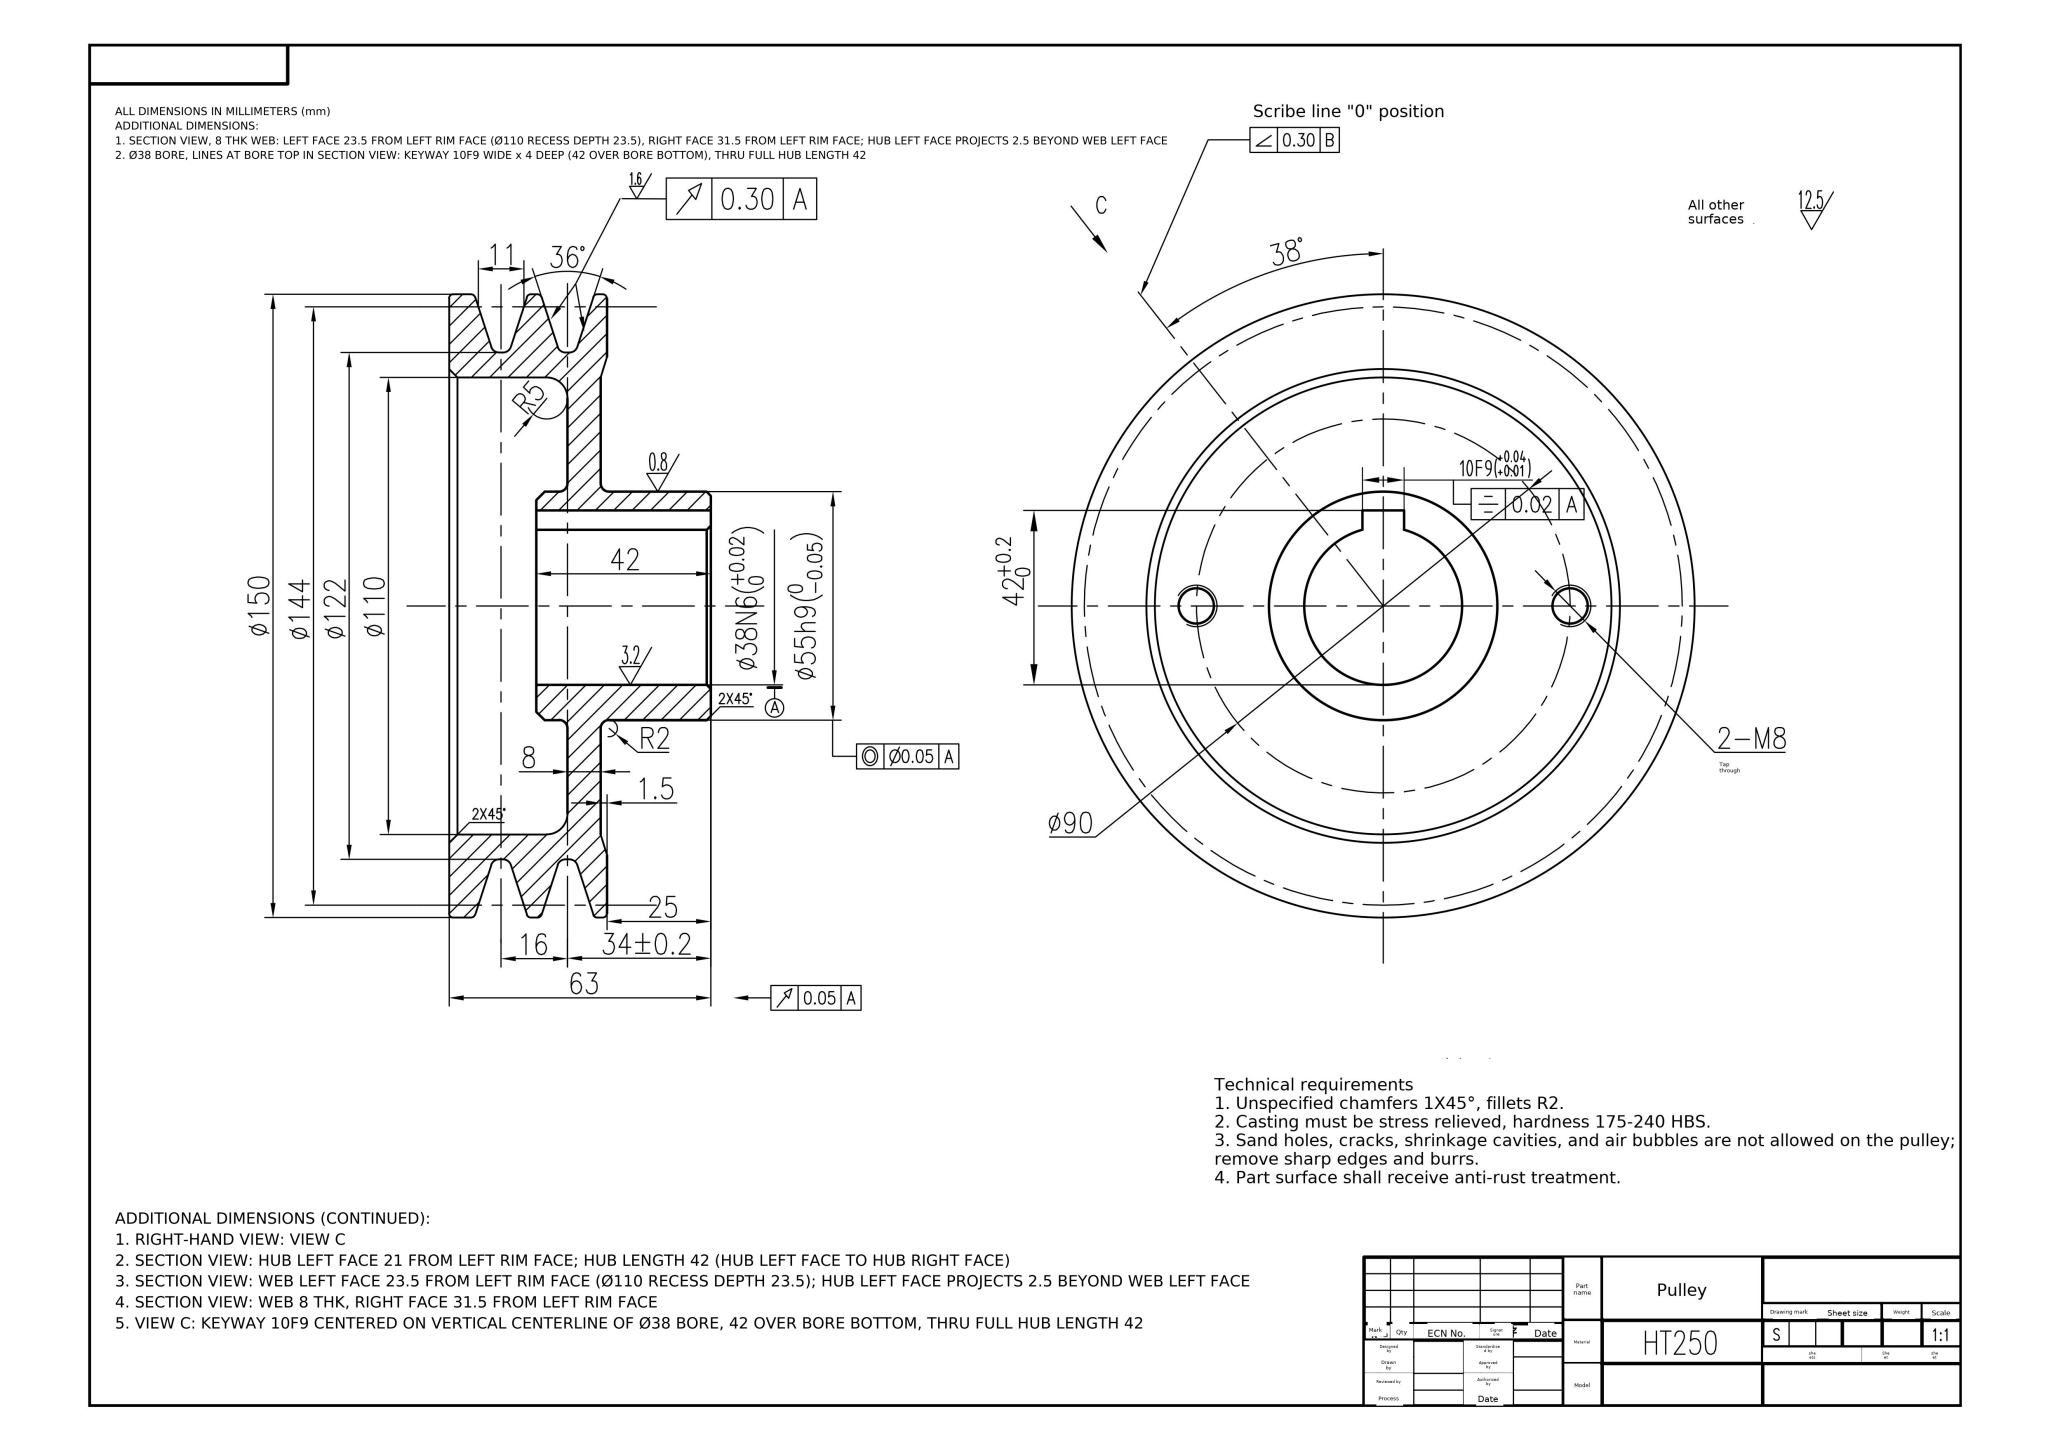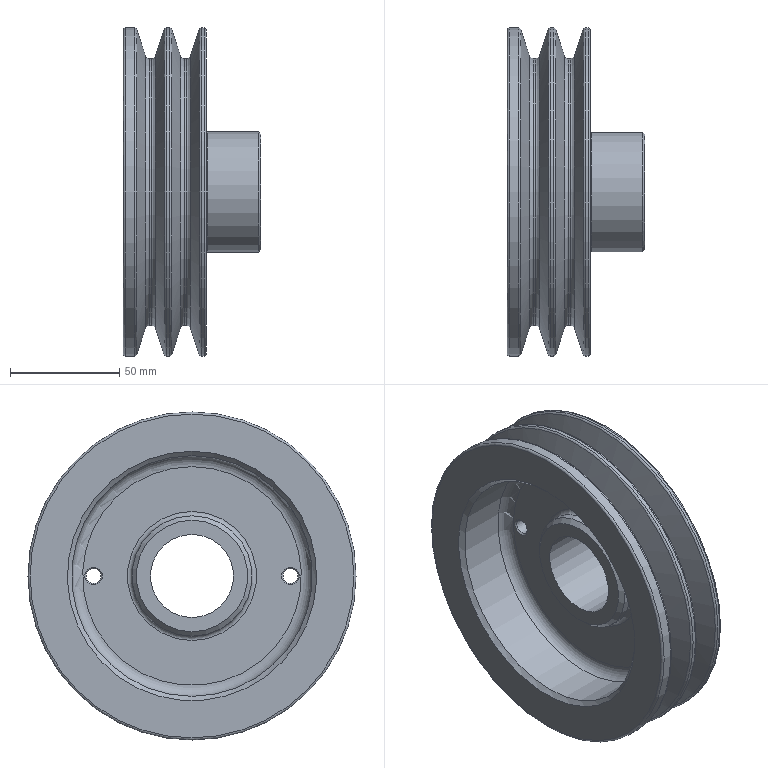Part | NX | mm | 1 solid | 43 faces | box 63 x 150 x 150 mm | volume 316417 mm3 | torus 13 | cone 13 | cylinder 11 | plane 6 | commonest cylinder face diameters 150 x3 122 x2 55 x2 6.8 x2 110 x1 38 x1
STEP:
#1=CARTESIAN_POINT('',(0.,0.,0.));
#2=DIRECTION('',(0.,0.,1.));
#3=DIRECTION('',(1.,0.,0.));
#4=AXIS2_PLACEMENT_3D('',#1,#2,#3);
#5=(LENGTH_UNIT()NAMED_UNIT(*)SI_UNIT(.MILLI.,.METRE.));
#6=UNCERTAINTY_MEASURE_WITH_UNIT(LENGTH_MEASURE(0.00002),#5,'','');
#7=(NAMED_UNIT(*)PLANE_ANGLE_UNIT()SI_UNIT($,.RADIAN.));
#8=PLANE_ANGLE_MEASURE_WITH_UNIT(PLANE_ANGLE_MEASURE(0.01745),#7);
#9=DIMENSIONAL_EXPONENTS(0.,0.,0.,0.,0.,0.,0.);
#10=(CONVERSION_BASED_UNIT('',#8)NAMED_UNIT(#9)PLANE_ANGLE_UNIT());
#11=(NAMED_UNIT(*)SI_UNIT($,.STERADIAN.)SOLID_ANGLE_UNIT());
#12=(GEOMETRIC_REPRESENTATION_CONTEXT(3)GLOBAL_UNCERTAINTY_ASSIGNED_CONTEXT((#6))GLOBAL_UNIT_ASSIGNED_CONTEXT((#5,#10,#11))REPRESENTATION_CONTEXT('',''));
#13=SHAPE_REPRESENTATION('',(#4),#12);
#14=CARTESIAN_POINT('',(-3947.497,-1111.045,29.5));
#15=VERTEX_POINT('',#14);
#16=CARTESIAN_POINT('',(-3947.497,-1111.045,0.));
#17=DIRECTION('',(-1.,0.,0.));
#18=DIRECTION('',(0.,0.,1.));
#19=AXIS2_PLACEMENT_3D('',#16,#17,#18);
#20=CIRCLE('',#19,29.5);
#21=EDGE_CURVE('',#15,#15,#20,.T.);
#22=ORIENTED_EDGE('',*,*,#21,.F.);
#23=EDGE_LOOP('',(#22));
#24=FACE_BOUND('',#23,.T.);
#25=CARTESIAN_POINT('',(-3945.497,-1111.045,27.5));
#26=VERTEX_POINT('',#25);
#27=CARTESIAN_POINT('',(-3945.497,-1111.045,0.));
#28=DIRECTION('',(-1.,0.,0.));
#29=DIRECTION('',(0.,0.,1.));
#30=AXIS2_PLACEMENT_3D('',#27,#28,#29);
#31=CIRCLE('',#30,27.5);
#32=EDGE_CURVE('',#26,#26,#31,.T.);
#33=ORIENTED_EDGE('',*,*,#32,.T.);
#34=EDGE_LOOP('',(#33));
#35=FACE_BOUND('',#34,.T.);
#36=CARTESIAN_POINT('',(-3945.497,-1111.045,0.));
#37=DIRECTION('',(-1.,0.,0.));
#38=DIRECTION('',(0.,0.,1.));
#39=AXIS2_PLACEMENT_3D('',#36,#37,#38);
#40=TOROIDAL_SURFACE('',#39,29.5,2.);
#41=ADVANCED_FACE('',(#24,#35),#40,.F.);
#42=CARTESIAN_POINT('',(-3947.497,-1156.045,4.));
#43=VERTEX_POINT('',#42);
#44=CARTESIAN_POINT('',(-3947.497,-1156.045,0.));
#45=DIRECTION('',(-1.,0.,0.));
#46=DIRECTION('',(0.,0.,1.));
#47=AXIS2_PLACEMENT_3D('',#44,#45,#46);
#48=CIRCLE('',#47,4.);
#49=EDGE_CURVE('',#43,#43,#48,.T.);
#50=ORIENTED_EDGE('',*,*,#49,.T.);
#51=EDGE_LOOP('',(#50));
#52=FACE_BOUND('',#51,.T.);
#53=CARTESIAN_POINT('',(-3947.497,-1066.045,4.));
#54=VERTEX_POINT('',#53);
#55=CARTESIAN_POINT('',(-3947.497,-1066.045,0.));
#56=DIRECTION('',(-1.,0.,0.));
#57=DIRECTION('',(0.,0.,1.));
#58=AXIS2_PLACEMENT_3D('',#55,#56,#57);
#59=CIRCLE('',#58,4.);
#60=EDGE_CURVE('',#54,#54,#59,.T.);
#61=ORIENTED_EDGE('',*,*,#60,.T.);
#62=EDGE_LOOP('',(#61));
#63=FACE_BOUND('',#62,.T.);
#64=CARTESIAN_POINT('',(-3947.497,-1111.045,55.));
#65=VERTEX_POINT('',#64);
#66=CARTESIAN_POINT('',(-3947.497,-1111.045,0.));
#67=DIRECTION('',(-1.,0.,0.));
#68=DIRECTION('',(0.,0.,1.));
#69=AXIS2_PLACEMENT_3D('',#66,#67,#68);
#70=CIRCLE('',#69,55.);
#71=EDGE_CURVE('',#65,#65,#70,.T.);
#72=ORIENTED_EDGE('',*,*,#71,.F.);
#73=EDGE_LOOP('',(#72));
#74=FACE_BOUND('',#73,.T.);
#75=ORIENTED_EDGE('',*,*,#21,.T.);
#76=EDGE_LOOP('',(#75));
#77=FACE_BOUND('',#76,.T.);
#78=CARTESIAN_POINT('',(-3947.497,-1140.545,0.));
#79=DIRECTION('',(-1.,0.,0.));
#80=DIRECTION('',(0.,0.,1.));
#81=AXIS2_PLACEMENT_3D('',#78,#79,#80);
#82=PLANE('',#81);
#83=ADVANCED_FACE('',(#52,#63,#74,#77),#82,.F.);
#84=CARTESIAN_POINT('',(-3945.997,-1111.045,60.));
#85=VERTEX_POINT('',#84);
#86=CARTESIAN_POINT('',(-3945.997,-1111.045,0.));
#87=DIRECTION('',(-1.,0.,0.));
#88=DIRECTION('',(0.,0.,1.));
#89=AXIS2_PLACEMENT_3D('',#86,#87,#88);
#90=CIRCLE('',#89,60.);
#91=EDGE_CURVE('',#85,#85,#90,.T.);
#92=ORIENTED_EDGE('',*,*,#91,.F.);
#93=EDGE_LOOP('',(#92));
#94=FACE_BOUND('',#93,.T.);
#95=ORIENTED_EDGE('',*,*,#71,.T.);
#96=EDGE_LOOP('',(#95));
#97=FACE_BOUND('',#96,.T.);
#98=CARTESIAN_POINT('',(-3947.497,-1111.045,0.));
#99=DIRECTION('',(1.,0.,0.));
#100=DIRECTION('',(0.,0.,-1.));
#101=AXIS2_PLACEMENT_3D('',#98,#99,#100);
#102=CONICAL_SURFACE('',#101,55.,73.301);
#103=ADVANCED_FACE('',(#94,#97),#102,.F.);
#104=CARTESIAN_POINT('',(-3945.997,-1111.045,74.));
#105=VERTEX_POINT('',#104);
#106=CARTESIAN_POINT('',(-3945.997,-1111.045,0.));
#107=DIRECTION('',(-1.,0.,0.));
#108=DIRECTION('',(0.,0.,1.));
#109=AXIS2_PLACEMENT_3D('',#106,#107,#108);
#110=CIRCLE('',#109,74.);
#111=EDGE_CURVE('',#105,#105,#110,.T.);
#112=ORIENTED_EDGE('',*,*,#111,.F.);
#113=EDGE_LOOP('',(#112));
#114=FACE_BOUND('',#113,.T.);
#115=ORIENTED_EDGE('',*,*,#91,.T.);
#116=EDGE_LOOP('',(#115));
#117=FACE_BOUND('',#116,.T.);
#118=CARTESIAN_POINT('',(-3945.997,-1171.045,0.));
#119=DIRECTION('',(-1.,0.,0.));
#120=DIRECTION('',(0.,0.,1.));
#121=AXIS2_PLACEMENT_3D('',#118,#119,#120);
#122=PLANE('',#121);
#123=ADVANCED_FACE('',(#114,#117),#122,.F.);
#124=CARTESIAN_POINT('',(-3946.997,-1111.045,75.));
#125=VERTEX_POINT('',#124);
#126=CARTESIAN_POINT('',(-3946.997,-1111.045,0.));
#127=DIRECTION('',(-1.,0.,0.));
#128=DIRECTION('',(0.,0.,1.));
#129=AXIS2_PLACEMENT_3D('',#126,#127,#128);
#130=CIRCLE('',#129,75.);
#131=EDGE_CURVE('',#125,#125,#130,.T.);
#132=ORIENTED_EDGE('',*,*,#131,.F.);
#133=EDGE_LOOP('',(#132));
#134=FACE_BOUND('',#133,.T.);
#135=ORIENTED_EDGE('',*,*,#111,.T.);
#136=EDGE_LOOP('',(#135));
#137=FACE_BOUND('',#136,.T.);
#138=CARTESIAN_POINT('',(-3946.997,-1111.045,0.));
#139=DIRECTION('',(-1.,0.,0.));
#140=DIRECTION('',(0.,0.,1.));
#141=AXIS2_PLACEMENT_3D('',#138,#139,#140);
#142=TOROIDAL_SURFACE('',#141,74.,1.);
#143=ADVANCED_FACE('',(#134,#137),#142,.T.);
#144=CARTESIAN_POINT('',(-3948.296,-1111.045,75.));
#145=VERTEX_POINT('',#144);
#146=CARTESIAN_POINT('',(-3948.296,-1111.045,0.));
#147=DIRECTION('',(-1.,0.,0.));
#148=DIRECTION('',(0.,0.,1.));
#149=AXIS2_PLACEMENT_3D('',#146,#147,#148);
#150=CIRCLE('',#149,75.);
#151=EDGE_CURVE('',#145,#145,#150,.T.);
#152=ORIENTED_EDGE('',*,*,#151,.F.);
#153=EDGE_LOOP('',(#152));
#154=FACE_BOUND('',#153,.T.);
#155=ORIENTED_EDGE('',*,*,#131,.T.);
#156=EDGE_LOOP('',(#155));
#157=FACE_BOUND('',#156,.T.);
#158=CARTESIAN_POINT('',(-3951.186,-1111.045,0.));
#159=DIRECTION('',(-1.,0.,0.));
#160=DIRECTION('',(0.,0.,1.));
#161=AXIS2_PLACEMENT_3D('',#158,#159,#160);
#162=CYLINDRICAL_SURFACE('',#161,75.);
#163=ADVANCED_FACE('',(#154,#157),#162,.T.);
#164=CARTESIAN_POINT('',(-3949.247,-1111.045,74.309));
#165=VERTEX_POINT('',#164);
#166=CARTESIAN_POINT('',(-3949.247,-1111.045,0.));
#167=DIRECTION('',(-1.,0.,0.));
#168=DIRECTION('',(0.,0.,1.));
#169=AXIS2_PLACEMENT_3D('',#166,#167,#168);
#170=CIRCLE('',#169,74.309);
#171=EDGE_CURVE('',#165,#165,#170,.T.);
#172=ORIENTED_EDGE('',*,*,#171,.F.);
#173=EDGE_LOOP('',(#172));
#174=FACE_BOUND('',#173,.T.);
#175=ORIENTED_EDGE('',*,*,#151,.T.);
#176=EDGE_LOOP('',(#175));
#177=FACE_BOUND('',#176,.T.);
#178=CARTESIAN_POINT('',(-3948.296,-1111.045,0.));
#179=DIRECTION('',(-1.,0.,0.));
#180=DIRECTION('',(0.,0.,1.));
#181=AXIS2_PLACEMENT_3D('',#178,#179,#180);
#182=TOROIDAL_SURFACE('',#181,74.,1.);
#183=ADVANCED_FACE('',(#174,#177),#182,.T.);
#184=CARTESIAN_POINT('',(-3953.122,-1111.045,62.382));
#185=VERTEX_POINT('',#184);
#186=CARTESIAN_POINT('',(-3953.122,-1111.045,0.));
#187=DIRECTION('',(-1.,0.,0.));
#188=DIRECTION('',(0.,0.,1.));
#189=AXIS2_PLACEMENT_3D('',#186,#187,#188);
#190=CIRCLE('',#189,62.382);
#191=EDGE_CURVE('',#185,#185,#190,.T.);
#192=ORIENTED_EDGE('',*,*,#191,.F.);
#193=EDGE_LOOP('',(#192));
#194=FACE_BOUND('',#193,.T.);
#195=ORIENTED_EDGE('',*,*,#171,.T.);
#196=EDGE_LOOP('',(#195));
#197=FACE_BOUND('',#196,.T.);
#198=CARTESIAN_POINT('',(-3949.247,-1111.045,0.));
#199=DIRECTION('',(1.,0.,0.));
#200=DIRECTION('',(0.,0.,-1.));
#201=AXIS2_PLACEMENT_3D('',#198,#199,#200);
#202=CONICAL_SURFACE('',#201,74.309,72.);
#203=ADVANCED_FACE('',(#194,#197),#202,.T.);
#204=CARTESIAN_POINT('',(-3955.024,-1111.045,61.));
#205=VERTEX_POINT('',#204);
#206=CARTESIAN_POINT('',(-3955.024,-1111.045,0.));
#207=DIRECTION('',(-1.,0.,0.));
#208=DIRECTION('',(0.,0.,1.));
#209=AXIS2_PLACEMENT_3D('',#206,#207,#208);
#210=CIRCLE('',#209,61.);
#211=EDGE_CURVE('',#205,#205,#210,.T.);
#212=ORIENTED_EDGE('',*,*,#211,.F.);
#213=EDGE_LOOP('',(#212));
#214=FACE_BOUND('',#213,.T.);
#215=ORIENTED_EDGE('',*,*,#191,.T.);
#216=EDGE_LOOP('',(#215));
#217=FACE_BOUND('',#216,.T.);
#218=CARTESIAN_POINT('',(-3955.024,-1111.045,0.));
#219=DIRECTION('',(-1.,0.,0.));
#220=DIRECTION('',(0.,0.,1.));
#221=AXIS2_PLACEMENT_3D('',#218,#219,#220);
#222=TOROIDAL_SURFACE('',#221,63.,2.);
#223=ADVANCED_FACE('',(#214,#217),#222,.F.);
#224=CARTESIAN_POINT('',(-3955.97,-1111.045,61.));
#225=VERTEX_POINT('',#224);
#226=CARTESIAN_POINT('',(-3955.97,-1111.045,0.));
#227=DIRECTION('',(-1.,0.,0.));
#228=DIRECTION('',(0.,0.,1.));
#229=AXIS2_PLACEMENT_3D('',#226,#227,#228);
#230=CIRCLE('',#229,61.);
#231=EDGE_CURVE('',#225,#225,#230,.T.);
#232=ORIENTED_EDGE('',*,*,#231,.F.);
#233=EDGE_LOOP('',(#232));
#234=FACE_BOUND('',#233,.T.);
#235=ORIENTED_EDGE('',*,*,#211,.T.);
#236=EDGE_LOOP('',(#235));
#237=FACE_BOUND('',#236,.T.);
#238=CARTESIAN_POINT('',(-3951.186,-1111.045,0.));
#239=DIRECTION('',(-1.,0.,0.));
#240=DIRECTION('',(0.,0.,1.));
#241=AXIS2_PLACEMENT_3D('',#238,#239,#240);
#242=CYLINDRICAL_SURFACE('',#241,61.);
#243=ADVANCED_FACE('',(#234,#237),#242,.T.);
#244=CARTESIAN_POINT('',(-3957.872,-1111.045,62.382));
#245=VERTEX_POINT('',#244);
#246=CARTESIAN_POINT('',(-3957.872,-1111.045,0.));
#247=DIRECTION('',(-1.,0.,0.));
#248=DIRECTION('',(0.,0.,1.));
#249=AXIS2_PLACEMENT_3D('',#246,#247,#248);
#250=CIRCLE('',#249,62.382);
#251=EDGE_CURVE('',#245,#245,#250,.T.);
#252=ORIENTED_EDGE('',*,*,#251,.F.);
#253=EDGE_LOOP('',(#252));
#254=FACE_BOUND('',#253,.T.);
#255=ORIENTED_EDGE('',*,*,#231,.T.);
#256=EDGE_LOOP('',(#255));
#257=FACE_BOUND('',#256,.T.);
#258=CARTESIAN_POINT('',(-3955.97,-1111.045,0.));
#259=DIRECTION('',(-1.,0.,0.));
#260=DIRECTION('',(0.,0.,1.));
#261=AXIS2_PLACEMENT_3D('',#258,#259,#260);
#262=TOROIDAL_SURFACE('',#261,63.,2.);
#263=ADVANCED_FACE('',(#254,#257),#262,.F.);
#264=CARTESIAN_POINT('',(-3961.747,-1111.045,74.309));
#265=VERTEX_POINT('',#264);
#266=CARTESIAN_POINT('',(-3961.747,-1111.045,0.));
#267=DIRECTION('',(-1.,0.,0.));
#268=DIRECTION('',(0.,0.,1.));
#269=AXIS2_PLACEMENT_3D('',#266,#267,#268);
#270=CIRCLE('',#269,74.309);
#271=EDGE_CURVE('',#265,#265,#270,.T.);
#272=ORIENTED_EDGE('',*,*,#271,.F.);
#273=EDGE_LOOP('',(#272));
#274=FACE_BOUND('',#273,.T.);
#275=ORIENTED_EDGE('',*,*,#251,.T.);
#276=EDGE_LOOP('',(#275));
#277=FACE_BOUND('',#276,.T.);
#278=CARTESIAN_POINT('',(-3957.872,-1111.045,0.));
#279=DIRECTION('',(-1.,0.,0.));
#280=DIRECTION('',(0.,0.,1.));
#281=AXIS2_PLACEMENT_3D('',#278,#279,#280);
#282=CONICAL_SURFACE('',#281,62.382,72.);
#283=ADVANCED_FACE('',(#274,#277),#282,.T.);
#284=CARTESIAN_POINT('',(-3962.698,-1111.045,75.));
#285=VERTEX_POINT('',#284);
#286=CARTESIAN_POINT('',(-3962.698,-1111.045,0.));
#287=DIRECTION('',(-1.,0.,0.));
#288=DIRECTION('',(0.,0.,1.));
#289=AXIS2_PLACEMENT_3D('',#286,#287,#288);
#290=CIRCLE('',#289,75.);
#291=EDGE_CURVE('',#285,#285,#290,.T.);
#292=ORIENTED_EDGE('',*,*,#291,.F.);
#293=EDGE_LOOP('',(#292));
#294=FACE_BOUND('',#293,.T.);
#295=ORIENTED_EDGE('',*,*,#271,.T.);
#296=EDGE_LOOP('',(#295));
#297=FACE_BOUND('',#296,.T.);
#298=CARTESIAN_POINT('',(-3962.698,-1111.045,0.));
#299=DIRECTION('',(-1.,0.,0.));
#300=DIRECTION('',(0.,0.,1.));
#301=AXIS2_PLACEMENT_3D('',#298,#299,#300);
#302=TOROIDAL_SURFACE('',#301,74.,1.);
#303=ADVANCED_FACE('',(#294,#297),#302,.T.);
#304=CARTESIAN_POINT('',(-3964.296,-1111.045,75.));
#305=VERTEX_POINT('',#304);
#306=CARTESIAN_POINT('',(-3964.296,-1111.045,0.));
#307=DIRECTION('',(-1.,0.,0.));
#308=DIRECTION('',(0.,0.,1.));
#309=AXIS2_PLACEMENT_3D('',#306,#307,#308);
#310=CIRCLE('',#309,75.);
#311=EDGE_CURVE('',#305,#305,#310,.T.);
#312=ORIENTED_EDGE('',*,*,#311,.F.);
#313=EDGE_LOOP('',(#312));
#314=FACE_BOUND('',#313,.T.);
#315=ORIENTED_EDGE('',*,*,#291,.T.);
#316=EDGE_LOOP('',(#315));
#317=FACE_BOUND('',#316,.T.);
#318=CARTESIAN_POINT('',(-3951.186,-1111.045,0.));
#319=DIRECTION('',(-1.,0.,0.));
#320=DIRECTION('',(0.,0.,1.));
#321=AXIS2_PLACEMENT_3D('',#318,#319,#320);
#322=CYLINDRICAL_SURFACE('',#321,75.);
#323=ADVANCED_FACE('',(#314,#317),#322,.T.);
#324=CARTESIAN_POINT('',(-3965.247,-1111.045,74.309));
#325=VERTEX_POINT('',#324);
#326=CARTESIAN_POINT('',(-3965.247,-1111.045,0.));
#327=DIRECTION('',(-1.,0.,0.));
#328=DIRECTION('',(0.,0.,1.));
#329=AXIS2_PLACEMENT_3D('',#326,#327,#328);
#330=CIRCLE('',#329,74.309);
#331=EDGE_CURVE('',#325,#325,#330,.T.);
#332=ORIENTED_EDGE('',*,*,#331,.F.);
#333=EDGE_LOOP('',(#332));
#334=FACE_BOUND('',#333,.T.);
#335=ORIENTED_EDGE('',*,*,#311,.T.);
#336=EDGE_LOOP('',(#335));
#337=FACE_BOUND('',#336,.T.);
#338=CARTESIAN_POINT('',(-3964.296,-1111.045,0.));
#339=DIRECTION('',(-1.,0.,0.));
#340=DIRECTION('',(0.,0.,1.));
#341=AXIS2_PLACEMENT_3D('',#338,#339,#340);
#342=TOROIDAL_SURFACE('',#341,74.,1.);
#343=ADVANCED_FACE('',(#334,#337),#342,.T.);
#344=CARTESIAN_POINT('',(-3969.122,-1111.045,62.382));
#345=VERTEX_POINT('',#344);
#346=CARTESIAN_POINT('',(-3969.122,-1111.045,0.));
#347=DIRECTION('',(-1.,0.,0.));
#348=DIRECTION('',(0.,0.,1.));
#349=AXIS2_PLACEMENT_3D('',#346,#347,#348);
#350=CIRCLE('',#349,62.382);
#351=EDGE_CURVE('',#345,#345,#350,.T.);
#352=ORIENTED_EDGE('',*,*,#351,.F.);
#353=EDGE_LOOP('',(#352));
#354=FACE_BOUND('',#353,.T.);
#355=ORIENTED_EDGE('',*,*,#331,.T.);
#356=EDGE_LOOP('',(#355));
#357=FACE_BOUND('',#356,.T.);
#358=CARTESIAN_POINT('',(-3965.247,-1111.045,0.));
#359=DIRECTION('',(1.,0.,0.));
#360=DIRECTION('',(0.,0.,-1.));
#361=AXIS2_PLACEMENT_3D('',#358,#359,#360);
#362=CONICAL_SURFACE('',#361,74.309,72.);
#363=ADVANCED_FACE('',(#354,#357),#362,.T.);
#364=CARTESIAN_POINT('',(-3971.024,-1111.045,61.));
#365=VERTEX_POINT('',#364);
#366=CARTESIAN_POINT('',(-3971.024,-1111.045,0.));
#367=DIRECTION('',(-1.,0.,0.));
#368=DIRECTION('',(0.,0.,1.));
#369=AXIS2_PLACEMENT_3D('',#366,#367,#368);
#370=CIRCLE('',#369,61.);
#371=EDGE_CURVE('',#365,#365,#370,.T.);
#372=ORIENTED_EDGE('',*,*,#371,.F.);
#373=EDGE_LOOP('',(#372));
#374=FACE_BOUND('',#373,.T.);
#375=ORIENTED_EDGE('',*,*,#351,.T.);
#376=EDGE_LOOP('',(#375));
#377=FACE_BOUND('',#376,.T.);
#378=CARTESIAN_POINT('',(-3971.024,-1111.045,0.));
#379=DIRECTION('',(-1.,0.,0.));
#380=DIRECTION('',(0.,0.,1.));
#381=AXIS2_PLACEMENT_3D('',#378,#379,#380);
#382=TOROIDAL_SURFACE('',#381,63.,2.);
#383=ADVANCED_FACE('',(#374,#377),#382,.F.);
#384=CARTESIAN_POINT('',(-3971.97,-1111.045,61.));
#385=VERTEX_POINT('',#384);
#386=CARTESIAN_POINT('',(-3971.97,-1111.045,0.));
#387=DIRECTION('',(-1.,0.,0.));
#388=DIRECTION('',(0.,0.,1.));
#389=AXIS2_PLACEMENT_3D('',#386,#387,#388);
#390=CIRCLE('',#389,61.);
#391=EDGE_CURVE('',#385,#385,#390,.T.);
#392=ORIENTED_EDGE('',*,*,#391,.F.);
#393=EDGE_LOOP('',(#392));
#394=FACE_BOUND('',#393,.T.);
#395=ORIENTED_EDGE('',*,*,#371,.T.);
#396=EDGE_LOOP('',(#395));
#397=FACE_BOUND('',#396,.T.);
#398=CARTESIAN_POINT('',(-3951.186,-1111.045,0.));
#399=DIRECTION('',(-1.,0.,0.));
#400=DIRECTION('',(0.,0.,1.));
#401=AXIS2_PLACEMENT_3D('',#398,#399,#400);
#402=CYLINDRICAL_SURFACE('',#401,61.);
#403=ADVANCED_FACE('',(#394,#397),#402,.T.);
#404=CARTESIAN_POINT('',(-3973.872,-1111.045,62.382));
#405=VERTEX_POINT('',#404);
#406=CARTESIAN_POINT('',(-3973.872,-1111.045,0.));
#407=DIRECTION('',(-1.,0.,0.));
#408=DIRECTION('',(0.,0.,1.));
#409=AXIS2_PLACEMENT_3D('',#406,#407,#408);
#410=CIRCLE('',#409,62.382);
#411=EDGE_CURVE('',#405,#405,#410,.T.);
#412=ORIENTED_EDGE('',*,*,#411,.F.);
#413=EDGE_LOOP('',(#412));
#414=FACE_BOUND('',#413,.T.);
#415=ORIENTED_EDGE('',*,*,#391,.T.);
#416=EDGE_LOOP('',(#415));
#417=FACE_BOUND('',#416,.T.);
#418=CARTESIAN_POINT('',(-3971.97,-1111.045,0.));
#419=DIRECTION('',(-1.,0.,0.));
#420=DIRECTION('',(0.,0.,1.));
#421=AXIS2_PLACEMENT_3D('',#418,#419,#420);
#422=TOROIDAL_SURFACE('',#421,63.,2.);
#423=ADVANCED_FACE('',(#414,#417),#422,.F.);
#424=CARTESIAN_POINT('',(-3977.747,-1111.045,74.309));
#425=VERTEX_POINT('',#424);
#426=CARTESIAN_POINT('',(-3977.747,-1111.045,0.));
#427=DIRECTION('',(-1.,0.,0.));
#428=DIRECTION('',(0.,0.,1.));
#429=AXIS2_PLACEMENT_3D('',#426,#427,#428);
#430=CIRCLE('',#429,74.309);
#431=EDGE_CURVE('',#425,#425,#430,.T.);
#432=ORIENTED_EDGE('',*,*,#431,.F.);
#433=EDGE_LOOP('',(#432));
#434=FACE_BOUND('',#433,.T.);
#435=ORIENTED_EDGE('',*,*,#411,.T.);
#436=EDGE_LOOP('',(#435));
#437=FACE_BOUND('',#436,.T.);
#438=CARTESIAN_POINT('',(-3973.872,-1111.045,0.));
#439=DIRECTION('',(-1.,0.,0.));
#440=DIRECTION('',(0.,0.,1.));
#441=AXIS2_PLACEMENT_3D('',#438,#439,#440);
#442=CONICAL_SURFACE('',#441,62.382,72.);
#443=ADVANCED_FACE('',(#434,#437),#442,.T.);
#444=CARTESIAN_POINT('',(-3978.698,-1111.045,75.));
#445=VERTEX_POINT('',#444);
#446=CARTESIAN_POINT('',(-3978.698,-1111.045,0.));
#447=DIRECTION('',(-1.,0.,0.));
#448=DIRECTION('',(0.,0.,1.));
#449=AXIS2_PLACEMENT_3D('',#446,#447,#448);
#450=CIRCLE('',#449,75.);
#451=EDGE_CURVE('',#445,#445,#450,.T.);
#452=ORIENTED_EDGE('',*,*,#451,.F.);
#453=EDGE_LOOP('',(#452));
#454=FACE_BOUND('',#453,.T.);
#455=ORIENTED_EDGE('',*,*,#431,.T.);
#456=EDGE_LOOP('',(#455));
#457=FACE_BOUND('',#456,.T.);
#458=CARTESIAN_POINT('',(-3978.698,-1111.045,0.));
#459=DIRECTION('',(-1.,0.,0.));
#460=DIRECTION('',(0.,0.,1.));
#461=AXIS2_PLACEMENT_3D('',#458,#459,#460);
#462=TOROIDAL_SURFACE('',#461,74.,1.);
#463=ADVANCED_FACE('',(#454,#457),#462,.T.);
#464=CARTESIAN_POINT('',(-3982.997,-1111.045,75.));
#465=VERTEX_POINT('',#464);
#466=CARTESIAN_POINT('',(-3982.997,-1111.045,0.));
#467=DIRECTION('',(-1.,0.,0.));
#468=DIRECTION('',(0.,0.,1.));
#469=AXIS2_PLACEMENT_3D('',#466,#467,#468);
#470=CIRCLE('',#469,75.);
#471=EDGE_CURVE('',#465,#465,#470,.T.);
#472=ORIENTED_EDGE('',*,*,#471,.F.);
#473=EDGE_LOOP('',(#472));
#474=FACE_BOUND('',#473,.T.);
#475=ORIENTED_EDGE('',*,*,#451,.T.);
#476=EDGE_LOOP('',(#475));
#477=FACE_BOUND('',#476,.T.);
#478=CARTESIAN_POINT('',(-3951.186,-1111.045,0.));
#479=DIRECTION('',(-1.,0.,0.));
#480=DIRECTION('',(0.,0.,1.));
#481=AXIS2_PLACEMENT_3D('',#478,#479,#480);
#482=CYLINDRICAL_SURFACE('',#481,75.);
#483=ADVANCED_FACE('',(#474,#477),#482,.T.);
#484=CARTESIAN_POINT('',(-3983.997,-1111.045,74.));
#485=VERTEX_POINT('',#484);
#486=CARTESIAN_POINT('',(-3983.997,-1111.045,0.));
#487=DIRECTION('',(-1.,0.,0.));
#488=DIRECTION('',(0.,0.,1.));
#489=AXIS2_PLACEMENT_3D('',#486,#487,#488);
#490=CIRCLE('',#489,74.);
#491=EDGE_CURVE('',#485,#485,#490,.T.);
#492=ORIENTED_EDGE('',*,*,#491,.F.);
#493=EDGE_LOOP('',(#492));
#494=FACE_BOUND('',#493,.T.);
#495=ORIENTED_EDGE('',*,*,#471,.T.);
#496=EDGE_LOOP('',(#495));
#497=FACE_BOUND('',#496,.T.);
#498=CARTESIAN_POINT('',(-3982.997,-1111.045,0.));
#499=DIRECTION('',(-1.,0.,0.));
#500=DIRECTION('',(0.,0.,1.));
#501=AXIS2_PLACEMENT_3D('',#498,#499,#500);
#502=TOROIDAL_SURFACE('',#501,74.,1.);
#503=ADVANCED_FACE('',(#494,#497),#502,.T.);
#504=CARTESIAN_POINT('',(-3983.997,-1111.045,57.));
#505=VERTEX_POINT('',#504);
#506=CARTESIAN_POINT('',(-3983.997,-1111.045,0.));
#507=DIRECTION('',(-1.,0.,0.));
#508=DIRECTION('',(0.,0.,1.));
#509=AXIS2_PLACEMENT_3D('',#506,#507,#508);
#510=CIRCLE('',#509,57.);
#511=EDGE_CURVE('',#505,#505,#510,.T.);
#512=ORIENTED_EDGE('',*,*,#511,.F.);
#513=EDGE_LOOP('',(#512));
#514=FACE_BOUND('',#513,.T.);
#515=ORIENTED_EDGE('',*,*,#491,.T.);
#516=EDGE_LOOP('',(#515));
#517=FACE_BOUND('',#516,.T.);
#518=CARTESIAN_POINT('',(-3983.997,-1185.045,0.));
#519=DIRECTION('',(1.,0.,0.));
#520=DIRECTION('',(0.,0.,-1.));
#521=AXIS2_PLACEMENT_3D('',#518,#519,#520);
#522=PLANE('',#521);
#523=ADVANCED_FACE('',(#514,#517),#522,.F.);
#524=CARTESIAN_POINT('',(-3981.997,-1111.045,55.));
#525=VERTEX_POINT('',#524);
#526=CARTESIAN_POINT('',(-3981.997,-1111.045,0.));
#527=DIRECTION('',(-1.,0.,0.));
#528=DIRECTION('',(0.,0.,1.));
#529=AXIS2_PLACEMENT_3D('',#526,#527,#528);
#530=CIRCLE('',#529,55.);
#531=EDGE_CURVE('',#525,#525,#530,.T.);
#532=ORIENTED_EDGE('',*,*,#531,.F.);
#533=EDGE_LOOP('',(#532));
#534=FACE_BOUND('',#533,.T.);
#535=ORIENTED_EDGE('',*,*,#511,.T.);
#536=EDGE_LOOP('',(#535));
#537=FACE_BOUND('',#536,.T.);
#538=CARTESIAN_POINT('',(-3983.997,-1111.045,0.));
#539=DIRECTION('',(-1.,0.,0.));
#540=DIRECTION('',(0.,0.,1.));
#541=AXIS2_PLACEMENT_3D('',#538,#539,#540);
#542=CONICAL_SURFACE('',#541,57.,45.);
#543=ADVANCED_FACE('',(#534,#537),#542,.F.);
#544=CARTESIAN_POINT('',(-3960.497,-1111.045,55.));
#545=VERTEX_POINT('',#544);
#546=CARTESIAN_POINT('',(-3960.497,-1111.045,0.));
#547=DIRECTION('',(-1.,0.,0.));
#548=DIRECTION('',(0.,0.,1.));
#549=AXIS2_PLACEMENT_3D('',#546,#547,#548);
#550=CIRCLE('',#549,55.);
#551=EDGE_CURVE('',#545,#545,#550,.T.);
#552=ORIENTED_EDGE('',*,*,#551,.F.);
#553=EDGE_LOOP('',(#552));
#554=FACE_BOUND('',#553,.T.);
#555=ORIENTED_EDGE('',*,*,#531,.T.);
#556=EDGE_LOOP('',(#555));
#557=FACE_BOUND('',#556,.T.);
#558=CARTESIAN_POINT('',(-3951.186,-1111.045,0.));
#559=DIRECTION('',(-1.,0.,0.));
#560=DIRECTION('',(0.,0.,1.));
#561=AXIS2_PLACEMENT_3D('',#558,#559,#560);
#562=CYLINDRICAL_SURFACE('',#561,55.);
#563=ADVANCED_FACE('',(#554,#557),#562,.F.);
#564=CARTESIAN_POINT('',(-3955.497,-1111.045,50.));
#565=VERTEX_POINT('',#564);
#566=CARTESIAN_POINT('',(-3955.497,-1111.045,0.));
#567=DIRECTION('',(-1.,0.,0.));
#568=DIRECTION('',(0.,0.,1.));
#569=AXIS2_PLACEMENT_3D('',#566,#567,#568);
#570=CIRCLE('',#569,50.);
#571=EDGE_CURVE('',#565,#565,#570,.T.);
#572=ORIENTED_EDGE('',*,*,#571,.F.);
#573=EDGE_LOOP('',(#572));
#574=FACE_BOUND('',#573,.T.);
#575=ORIENTED_EDGE('',*,*,#551,.T.);
#576=EDGE_LOOP('',(#575));
#577=FACE_BOUND('',#576,.T.);
#578=CARTESIAN_POINT('',(-3960.497,-1111.045,0.));
#579=DIRECTION('',(-1.,0.,0.));
#580=DIRECTION('',(0.,0.,1.));
#581=AXIS2_PLACEMENT_3D('',#578,#579,#580);
#582=TOROIDAL_SURFACE('',#581,50.,5.);
#583=ADVANCED_FACE('',(#574,#577),#582,.F.);
#584=CARTESIAN_POINT('',(-3955.497,-1156.045,-4.));
#585=VERTEX_POINT('',#584);
#586=CARTESIAN_POINT('',(-3955.497,-1156.045,0.));
#587=DIRECTION('',(1.,0.,0.));
#588=DIRECTION('',(0.,0.,-1.));
#589=AXIS2_PLACEMENT_3D('',#586,#587,#588);
#590=CIRCLE('',#589,4.);
#591=EDGE_CURVE('',#585,#585,#590,.T.);
#592=ORIENTED_EDGE('',*,*,#591,.T.);
#593=EDGE_LOOP('',(#592));
#594=FACE_BOUND('',#593,.T.);
#595=CARTESIAN_POINT('',(-3955.497,-1066.045,-4.));
#596=VERTEX_POINT('',#595);
#597=CARTESIAN_POINT('',(-3955.497,-1066.045,0.));
#598=DIRECTION('',(1.,0.,0.));
#599=DIRECTION('',(0.,0.,-1.));
#600=AXIS2_PLACEMENT_3D('',#597,#598,#599);
#601=CIRCLE('',#600,4.);
#602=EDGE_CURVE('',#596,#596,#601,.T.);
#603=ORIENTED_EDGE('',*,*,#602,.T.);
#604=EDGE_LOOP('',(#603));
#605=FACE_BOUND('',#604,.T.);
#606=CARTESIAN_POINT('',(-3955.497,-1111.045,29.5));
#607=VERTEX_POINT('',#606);
#608=CARTESIAN_POINT('',(-3955.497,-1111.045,0.));
#609=DIRECTION('',(-1.,0.,0.));
#610=DIRECTION('',(0.,0.,1.));
#611=AXIS2_PLACEMENT_3D('',#608,#609,#610);
#612=CIRCLE('',#611,29.5);
#613=EDGE_CURVE('',#607,#607,#612,.T.);
#614=ORIENTED_EDGE('',*,*,#613,.F.);
#615=EDGE_LOOP('',(#614));
#616=FACE_BOUND('',#615,.T.);
#617=ORIENTED_EDGE('',*,*,#571,.T.);
#618=EDGE_LOOP('',(#617));
#619=FACE_BOUND('',#618,.T.);
#620=CARTESIAN_POINT('',(-3955.497,-1161.045,0.));
#621=DIRECTION('',(1.,0.,0.));
#622=DIRECTION('',(0.,0.,-1.));
#623=AXIS2_PLACEMENT_3D('',#620,#621,#622);
#624=PLANE('',#623);
#625=ADVANCED_FACE('',(#594,#605,#616,#619),#624,.F.);
#626=CARTESIAN_POINT('',(-3957.497,-1111.045,27.5));
#627=VERTEX_POINT('',#626);
#628=CARTESIAN_POINT('',(-3957.497,-1111.045,0.));
#629=DIRECTION('',(-1.,0.,0.));
#630=DIRECTION('',(0.,0.,1.));
#631=AXIS2_PLACEMENT_3D('',#628,#629,#630);
#632=CIRCLE('',#631,27.5);
#633=EDGE_CURVE('',#627,#627,#632,.T.);
#634=ORIENTED_EDGE('',*,*,#633,.F.);
#635=EDGE_LOOP('',(#634));
#636=FACE_BOUND('',#635,.T.);
#637=ORIENTED_EDGE('',*,*,#613,.T.);
#638=EDGE_LOOP('',(#637));
#639=FACE_BOUND('',#638,.T.);
#640=CARTESIAN_POINT('',(-3957.497,-1111.045,0.));
#641=DIRECTION('',(-1.,0.,0.));
#642=DIRECTION('',(0.,0.,1.));
#643=AXIS2_PLACEMENT_3D('',#640,#641,#642);
#644=TOROIDAL_SURFACE('',#643,29.5,2.);
#645=ADVANCED_FACE('',(#636,#639),#644,.F.);
#646=CARTESIAN_POINT('',(-3960.997,-1111.045,27.5));
#647=VERTEX_POINT('',#646);
#648=CARTESIAN_POINT('',(-3960.997,-1111.045,0.));
#649=DIRECTION('',(-1.,0.,0.));
#650=DIRECTION('',(0.,0.,1.));
#651=AXIS2_PLACEMENT_3D('',#648,#649,#650);
#652=CIRCLE('',#651,27.5);
#653=EDGE_CURVE('',#647,#647,#652,.T.);
#654=ORIENTED_EDGE('',*,*,#653,.F.);
#655=EDGE_LOOP('',(#654));
#656=FACE_BOUND('',#655,.T.);
#657=ORIENTED_EDGE('',*,*,#633,.T.);
#658=EDGE_LOOP('',(#657));
#659=FACE_BOUND('',#658,.T.);
#660=CARTESIAN_POINT('',(-3951.186,-1111.045,0.));
#661=DIRECTION('',(-1.,0.,0.));
#662=DIRECTION('',(0.,0.,1.));
#663=AXIS2_PLACEMENT_3D('',#660,#661,#662);
#664=CYLINDRICAL_SURFACE('',#663,27.5);
#665=ADVANCED_FACE('',(#656,#659),#664,.T.);
#666=CARTESIAN_POINT('',(-3962.997,-1111.045,25.5));
#667=VERTEX_POINT('',#666);
#668=CARTESIAN_POINT('',(-3962.997,-1111.045,0.));
#669=DIRECTION('',(-1.,0.,0.));
#670=DIRECTION('',(0.,0.,1.));
#671=AXIS2_PLACEMENT_3D('',#668,#669,#670);
#672=CIRCLE('',#671,25.5);
#673=EDGE_CURVE('',#667,#667,#672,.T.);
#674=ORIENTED_EDGE('',*,*,#673,.F.);
#675=EDGE_LOOP('',(#674));
#676=FACE_BOUND('',#675,.T.);
#677=ORIENTED_EDGE('',*,*,#653,.T.);
#678=EDGE_LOOP('',(#677));
#679=FACE_BOUND('',#678,.T.);
#680=CARTESIAN_POINT('',(-3960.997,-1111.045,0.));
#681=DIRECTION('',(1.,0.,0.));
#682=DIRECTION('',(0.,0.,-1.));
#683=AXIS2_PLACEMENT_3D('',#680,#681,#682);
#684=CONICAL_SURFACE('',#683,27.5,45.);
#685=ADVANCED_FACE('',(#676,#679),#684,.T.);
#686=CARTESIAN_POINT('',(-3962.997,-1111.045,19.));
#687=VERTEX_POINT('',#686);
#688=CARTESIAN_POINT('',(-3962.997,-1111.045,0.));
#689=DIRECTION('',(-1.,0.,0.));
#690=DIRECTION('',(0.,0.,1.));
#691=AXIS2_PLACEMENT_3D('',#688,#689,#690);
#692=CIRCLE('',#691,19.);
#693=EDGE_CURVE('',#687,#687,#692,.T.);
#694=ORIENTED_EDGE('',*,*,#693,.F.);
#695=EDGE_LOOP('',(#694));
#696=FACE_BOUND('',#695,.T.);
#697=ORIENTED_EDGE('',*,*,#673,.T.);
#698=EDGE_LOOP('',(#697));
#699=FACE_BOUND('',#698,.T.);
#700=CARTESIAN_POINT('',(-3962.997,-1136.545,0.));
#701=DIRECTION('',(1.,0.,0.));
#702=DIRECTION('',(0.,0.,-1.));
#703=AXIS2_PLACEMENT_3D('',#700,#701,#702);
#704=PLANE('',#703);
#705=ADVANCED_FACE('',(#696,#699),#704,.F.);
#706=CARTESIAN_POINT('',(-3921.997,-1111.045,19.));
#707=VERTEX_POINT('',#706);
#708=CARTESIAN_POINT('',(-3921.997,-1111.045,0.));
#709=DIRECTION('',(-1.,0.,0.));
#710=DIRECTION('',(0.,0.,1.));
#711=AXIS2_PLACEMENT_3D('',#708,#709,#710);
#712=CIRCLE('',#711,19.);
#713=EDGE_CURVE('',#707,#707,#712,.T.);
#714=ORIENTED_EDGE('',*,*,#713,.F.);
#715=EDGE_LOOP('',(#714));
#716=FACE_BOUND('',#715,.T.);
#717=ORIENTED_EDGE('',*,*,#693,.T.);
#718=EDGE_LOOP('',(#717));
#719=FACE_BOUND('',#718,.T.);
#720=CARTESIAN_POINT('',(-3951.186,-1111.045,0.));
#721=DIRECTION('',(-1.,0.,0.));
#722=DIRECTION('',(0.,0.,1.));
#723=AXIS2_PLACEMENT_3D('',#720,#721,#722);
#724=CYLINDRICAL_SURFACE('',#723,19.);
#725=ADVANCED_FACE('',(#716,#719),#724,.F.);
#726=CARTESIAN_POINT('',(-3920.997,-1111.045,20.005));
#727=VERTEX_POINT('',#726);
#728=CARTESIAN_POINT('',(-3920.997,-1111.045,0.));
#729=DIRECTION('',(-1.,0.,0.));
#730=DIRECTION('',(0.,0.,1.));
#731=AXIS2_PLACEMENT_3D('',#728,#729,#730);
#732=CIRCLE('',#731,20.005);
#733=EDGE_CURVE('',#727,#727,#732,.T.);
#734=ORIENTED_EDGE('',*,*,#733,.F.);
#735=EDGE_LOOP('',(#734));
#736=FACE_BOUND('',#735,.T.);
#737=ORIENTED_EDGE('',*,*,#713,.T.);
#738=EDGE_LOOP('',(#737));
#739=FACE_BOUND('',#738,.T.);
#740=CARTESIAN_POINT('',(-3921.997,-1111.045,0.));
#741=DIRECTION('',(1.,0.,0.));
#742=DIRECTION('',(0.,0.,-1.));
#743=AXIS2_PLACEMENT_3D('',#740,#741,#742);
#744=CONICAL_SURFACE('',#743,19.,45.146);
#745=ADVANCED_FACE('',(#736,#739),#744,.F.);
#746=CARTESIAN_POINT('',(-3920.997,-1111.045,26.503));
#747=VERTEX_POINT('',#746);
#748=CARTESIAN_POINT('',(-3920.997,-1111.045,0.));
#749=DIRECTION('',(-1.,0.,0.));
#750=DIRECTION('',(0.,0.,1.));
#751=AXIS2_PLACEMENT_3D('',#748,#749,#750);
#752=CIRCLE('',#751,26.503);
#753=EDGE_CURVE('',#747,#747,#752,.T.);
#754=ORIENTED_EDGE('',*,*,#753,.F.);
#755=EDGE_LOOP('',(#754));
#756=FACE_BOUND('',#755,.T.);
#757=ORIENTED_EDGE('',*,*,#733,.T.);
#758=EDGE_LOOP('',(#757));
#759=FACE_BOUND('',#758,.T.);
#760=CARTESIAN_POINT('',(-3920.997,-1131.05,0.));
#761=DIRECTION('',(-1.,0.,0.));
#762=DIRECTION('',(0.,0.,1.));
#763=AXIS2_PLACEMENT_3D('',#760,#761,#762);
#764=PLANE('',#763);
#765=ADVANCED_FACE('',(#756,#759),#764,.F.);
#766=CARTESIAN_POINT('',(-3921.997,-1111.045,27.5));
#767=VERTEX_POINT('',#766);
#768=CARTESIAN_POINT('',(-3921.997,-1111.045,0.));
#769=DIRECTION('',(-1.,0.,0.));
#770=DIRECTION('',(0.,0.,1.));
#771=AXIS2_PLACEMENT_3D('',#768,#769,#770);
#772=CIRCLE('',#771,27.5);
#773=EDGE_CURVE('',#767,#767,#772,.T.);
#774=ORIENTED_EDGE('',*,*,#773,.F.);
#775=EDGE_LOOP('',(#774));
#776=FACE_BOUND('',#775,.T.);
#777=ORIENTED_EDGE('',*,*,#753,.T.);
#778=EDGE_LOOP('',(#777));
#779=FACE_BOUND('',#778,.T.);
#780=CARTESIAN_POINT('',(-3920.997,-1111.045,0.));
#781=DIRECTION('',(-1.,0.,0.));
#782=DIRECTION('',(0.,0.,1.));
#783=AXIS2_PLACEMENT_3D('',#780,#781,#782);
#784=CONICAL_SURFACE('',#783,26.503,44.905);
#785=ADVANCED_FACE('',(#776,#779),#784,.T.);
#786=ORIENTED_EDGE('',*,*,#32,.F.);
#787=EDGE_LOOP('',(#786));
#788=FACE_BOUND('',#787,.T.);
#789=ORIENTED_EDGE('',*,*,#773,.T.);
#790=EDGE_LOOP('',(#789));
#791=FACE_BOUND('',#790,.T.);
#792=CARTESIAN_POINT('',(-3951.186,-1111.045,0.));
#793=DIRECTION('',(-1.,0.,0.));
#794=DIRECTION('',(0.,0.,1.));
#795=AXIS2_PLACEMENT_3D('',#792,#793,#794);
#796=CYLINDRICAL_SURFACE('',#795,27.5);
#797=ADVANCED_FACE('',(#788,#791),#796,.T.);
#798=CARTESIAN_POINT('',(-3948.097,-1066.045,3.4));
#799=VERTEX_POINT('',#798);
#800=CARTESIAN_POINT('',(-3948.097,-1066.045,0.));
#801=DIRECTION('',(1.,0.,0.));
#802=DIRECTION('',(0.,0.,1.));
#803=AXIS2_PLACEMENT_3D('',#800,#801,#802);
#804=CIRCLE('',#803,3.4);
#805=EDGE_CURVE('',#799,#799,#804,.T.);
#806=ORIENTED_EDGE('',*,*,#805,.T.);
#807=EDGE_LOOP('',(#806));
#808=FACE_BOUND('',#807,.T.);
#809=CARTESIAN_POINT('',(-3954.897,-1066.045,-3.4));
#810=VERTEX_POINT('',#809);
#811=CARTESIAN_POINT('',(-3954.897,-1066.045,0.));
#812=DIRECTION('',(-1.,0.,0.));
#813=DIRECTION('',(0.,0.,-1.));
#814=AXIS2_PLACEMENT_3D('',#811,#812,#813);
#815=CIRCLE('',#814,3.4);
#816=EDGE_CURVE('',#810,#810,#815,.T.);
#817=ORIENTED_EDGE('',*,*,#816,.T.);
#818=EDGE_LOOP('',(#817));
#819=FACE_BOUND('',#818,.T.);
#820=CARTESIAN_POINT('',(-3955.497,-1066.045,0.));
#821=DIRECTION('',(1.,0.,0.));
#822=DIRECTION('',(0.,0.,-1.));
#823=AXIS2_PLACEMENT_3D('',#820,#821,#822);
#824=CYLINDRICAL_SURFACE('',#823,3.4);
#825=ADVANCED_FACE('',(#808,#819),#824,.F.);
#826=ORIENTED_EDGE('',*,*,#816,.F.);
#827=EDGE_LOOP('',(#826));
#828=FACE_BOUND('',#827,.T.);
#829=ORIENTED_EDGE('',*,*,#602,.F.);
#830=EDGE_LOOP('',(#829));
#831=FACE_BOUND('',#830,.T.);
#832=CARTESIAN_POINT('',(-3955.497,-1066.045,0.));
#833=DIRECTION('',(-1.,0.,0.));
#834=DIRECTION('',(0.,0.,1.));
#835=AXIS2_PLACEMENT_3D('',#832,#833,#834);
#836=CONICAL_SURFACE('',#835,4.,45.);
#837=ADVANCED_FACE('',(#828,#831),#836,.F.);
#838=ORIENTED_EDGE('',*,*,#805,.F.);
#839=EDGE_LOOP('',(#838));
#840=FACE_BOUND('',#839,.T.);
#841=ORIENTED_EDGE('',*,*,#60,.F.);
#842=EDGE_LOOP('',(#841));
#843=FACE_BOUND('',#842,.T.);
#844=CARTESIAN_POINT('',(-3947.497,-1066.045,0.));
#845=DIRECTION('',(1.,0.,0.));
#846=DIRECTION('',(0.,0.,-1.));
#847=AXIS2_PLACEMENT_3D('',#844,#845,#846);
#848=CONICAL_SURFACE('',#847,4.,45.);
#849=ADVANCED_FACE('',(#840,#843),#848,.F.);
#850=CARTESIAN_POINT('',(-3948.097,-1156.045,3.4));
#851=VERTEX_POINT('',#850);
#852=CARTESIAN_POINT('',(-3948.097,-1156.045,0.));
#853=DIRECTION('',(1.,0.,0.));
#854=DIRECTION('',(0.,0.,1.));
#855=AXIS2_PLACEMENT_3D('',#852,#853,#854);
#856=CIRCLE('',#855,3.4);
#857=EDGE_CURVE('',#851,#851,#856,.T.);
#858=ORIENTED_EDGE('',*,*,#857,.T.);
#859=EDGE_LOOP('',(#858));
#860=FACE_BOUND('',#859,.T.);
#861=CARTESIAN_POINT('',(-3954.897,-1156.045,-3.4));
#862=VERTEX_POINT('',#861);
#863=CARTESIAN_POINT('',(-3954.897,-1156.045,0.));
#864=DIRECTION('',(-1.,0.,0.));
#865=DIRECTION('',(0.,0.,-1.));
#866=AXIS2_PLACEMENT_3D('',#863,#864,#865);
#867=CIRCLE('',#866,3.4);
#868=EDGE_CURVE('',#862,#862,#867,.T.);
#869=ORIENTED_EDGE('',*,*,#868,.T.);
#870=EDGE_LOOP('',(#869));
#871=FACE_BOUND('',#870,.T.);
#872=CARTESIAN_POINT('',(-3955.497,-1156.045,0.));
#873=DIRECTION('',(1.,0.,0.));
#874=DIRECTION('',(0.,0.,-1.));
#875=AXIS2_PLACEMENT_3D('',#872,#873,#874);
#876=CYLINDRICAL_SURFACE('',#875,3.4);
#877=ADVANCED_FACE('',(#860,#871),#876,.F.);
#878=ORIENTED_EDGE('',*,*,#868,.F.);
#879=EDGE_LOOP('',(#878));
#880=FACE_BOUND('',#879,.T.);
#881=ORIENTED_EDGE('',*,*,#591,.F.);
#882=EDGE_LOOP('',(#881));
#883=FACE_BOUND('',#882,.T.);
#884=CARTESIAN_POINT('',(-3955.497,-1156.045,0.));
#885=DIRECTION('',(-1.,0.,0.));
#886=DIRECTION('',(0.,0.,1.));
#887=AXIS2_PLACEMENT_3D('',#884,#885,#886);
#888=CONICAL_SURFACE('',#887,4.,45.);
#889=ADVANCED_FACE('',(#880,#883),#888,.F.);
#890=ORIENTED_EDGE('',*,*,#857,.F.);
#891=EDGE_LOOP('',(#890));
#892=FACE_BOUND('',#891,.T.);
#893=ORIENTED_EDGE('',*,*,#49,.F.);
#894=EDGE_LOOP('',(#893));
#895=FACE_BOUND('',#894,.T.);
#896=CARTESIAN_POINT('',(-3947.497,-1156.045,0.));
#897=DIRECTION('',(1.,0.,0.));
#898=DIRECTION('',(0.,0.,-1.));
#899=AXIS2_PLACEMENT_3D('',#896,#897,#898);
#900=CONICAL_SURFACE('',#899,4.,45.);
#901=ADVANCED_FACE('',(#892,#895),#900,.F.);
#902=CLOSED_SHELL('',(#41,#83,#103,#123,#143,#163,#183,#203,#223,#243,#263,#283,#303,#323,#343,#363,#383,#403,#423,#443,#463,#483,#503,#523,#543,#563,#583,#625,#645,#665,#685,#705,#725,#745,#765,#785,#797,#825,#837,#849,#877,#889,#901));
#903=MANIFOLD_SOLID_BREP('',#902);
#904=ADVANCED_BREP_SHAPE_REPRESENTATION('',(#903),#12);
#905=SHAPE_REPRESENTATION_RELATIONSHIP('','',#13,#904);
#906=PRESENTATION_LAYER_ASSIGNMENT('','',(#903));
#907=COLOUR_RGB('',0.5961,0.6667,0.6863);
#908=FILL_AREA_STYLE_COLOUR('',#907);
#909=FILL_AREA_STYLE('',(#908));
#910=SURFACE_STYLE_FILL_AREA(#909);
#911=SURFACE_SIDE_STYLE('',(#910));
#912=SURFACE_STYLE_USAGE(.BOTH.,#911);
#913=PRESENTATION_STYLE_ASSIGNMENT((#912));
#914=STYLED_ITEM('',(#913),#903);
#915=MECHANICAL_DESIGN_GEOMETRIC_PRESENTATION_REPRESENTATION('',(#914),#12);